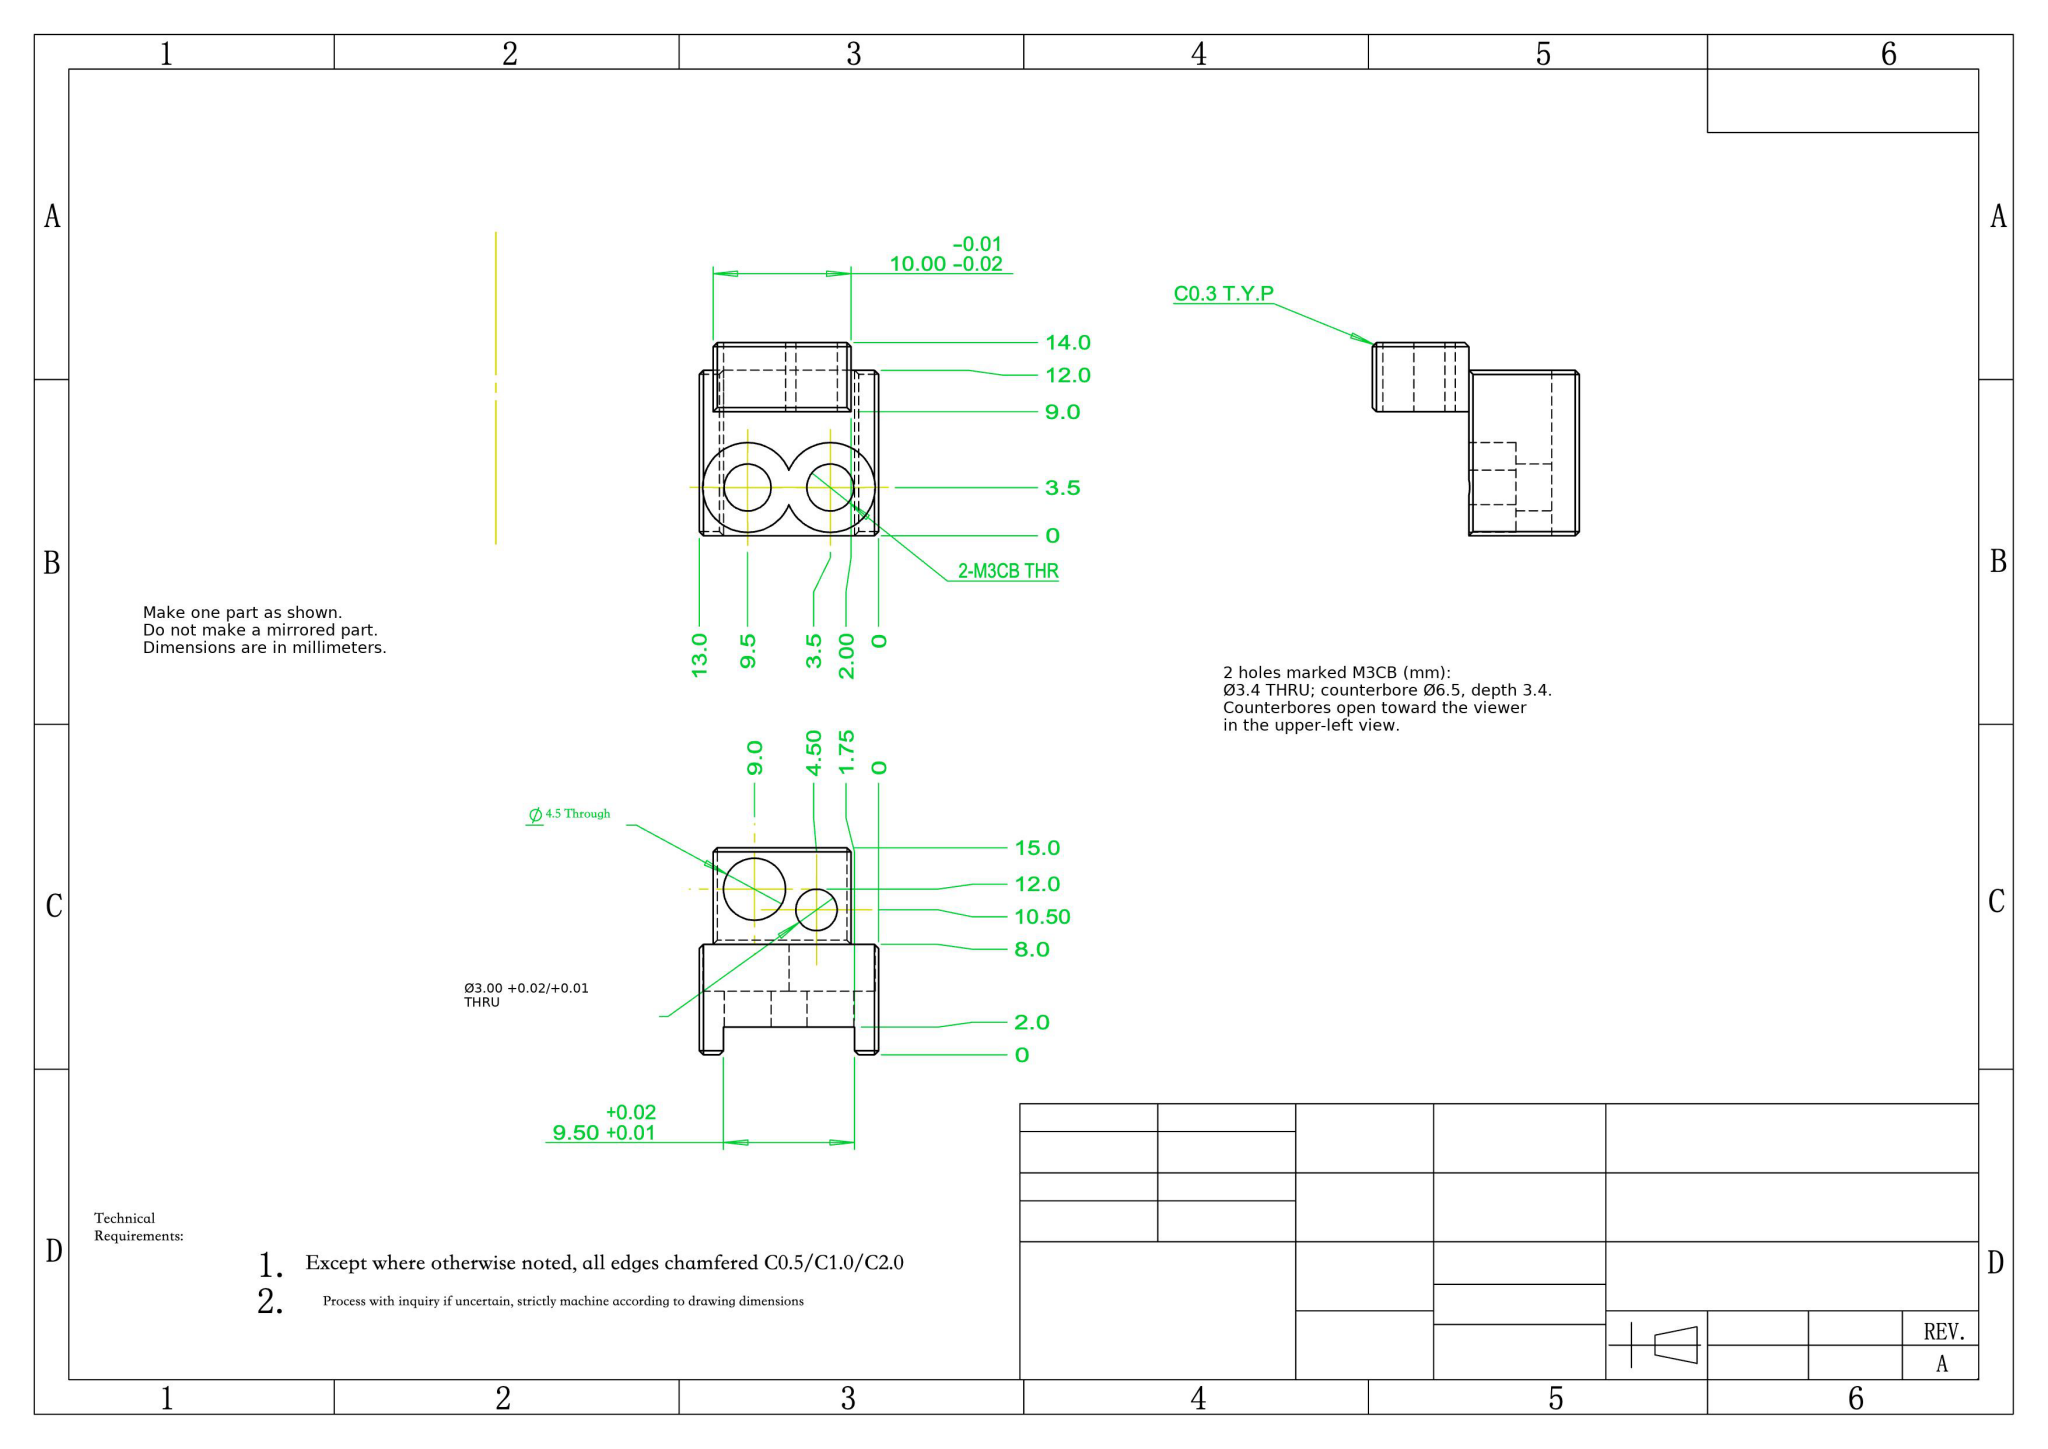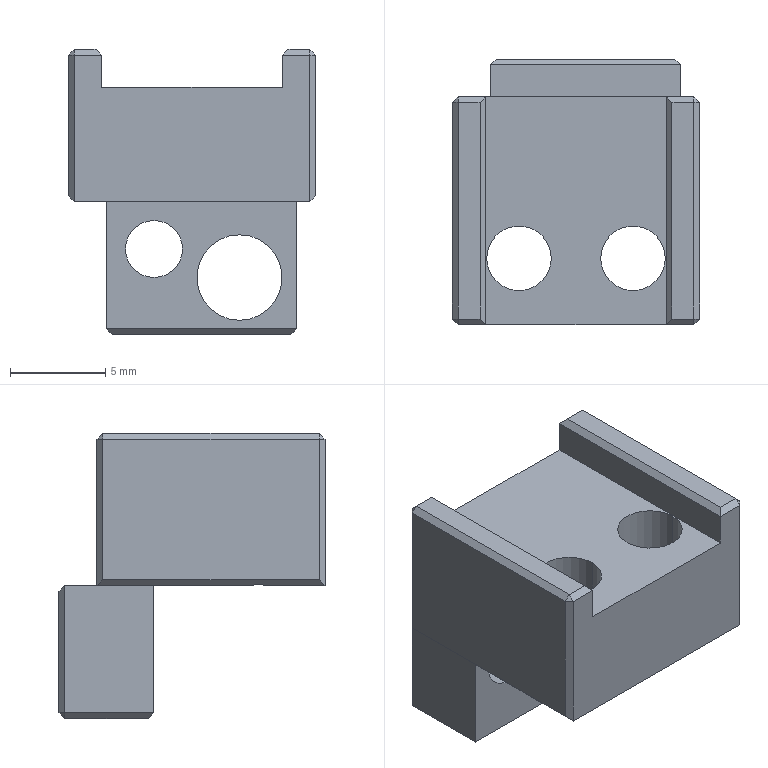Part | NX | mm | Stepped Multi-Bore Corner Mount | 1 solid | 56 faces | box 13 x 14 x 15 mm | volume 978 mm3 | plane 45 | cylinder 11 | commonest cylinder face diameters 3.4 x4 6.5 x3 3 x2 4.5 x2